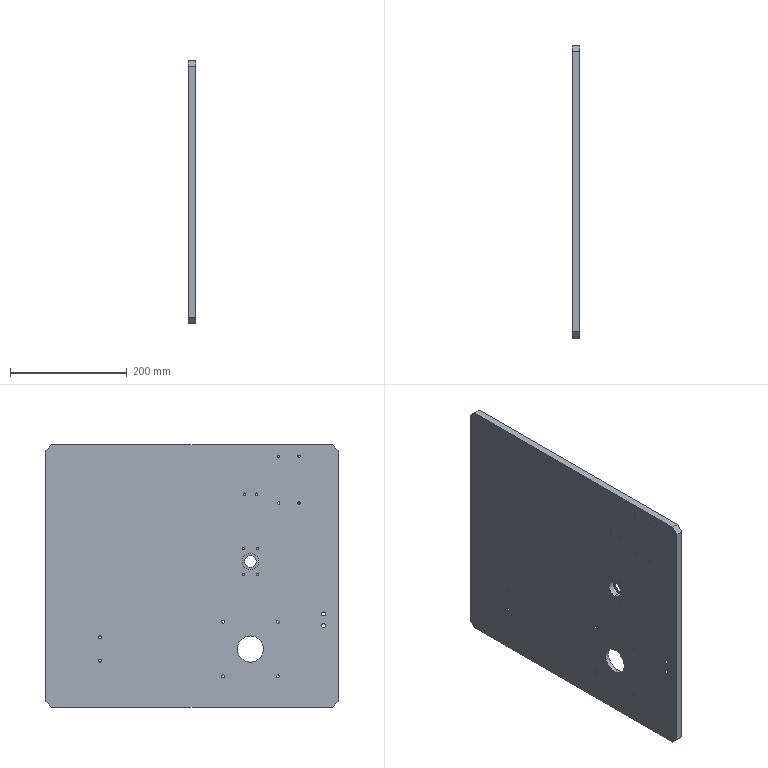Component | SolidWorks | ElectricalBoxAssembly2-1_Part6-1 | 1 solid | 56 faces | box 12 x 500 x 450 mm | volume 2647361 mm3 | cylinder 44 | plane 12 | commonest cylinder face diameters 4.2 x20 5 x12 6.8 x4 28 x2 85 x2 45 x2 20 x2
build123d program:
from build123d import *

# Parameters (mm, degrees)
SKETCH1_W            = 450
SKETCH1_H            = 500
SKETCH1_R            = 22.5
SKETCH1_R_2          = 10
BOSS_EXTRUDE1_DEPTH  = 12
M6_TAPPED_HOLE1_D    = 5
M5_TAPPED_HOLE1_D    = 4.2
M8_TAPPED_HOLE1_D    = 6.8
SKETCH9_R            = 42.5
CUT_EXTRUDE1_DEPTH   = 5
SKETCH10_R           = 14
CUT_EXTRUDE2_DEPTH   = 10
M5_TAPPED_HOLE2_D    = 4.2
M6_TAPPED_HOLE2_D    = 5
LPATTERN1_COUNT      = 2
LPATTERN1_PITCH      = 24
LPATTERN1_COUNT_DIR2 = 2
LPATTERN1_PITCH_DIR2 = 44
CHAMFER1_SIZE        = 10


with BuildPart() as part:
    # Sketch1 → Boss-Extrude1 (new body)
    with BuildSketch(Plane.XY):
        Rectangle(SKETCH1_W, SKETCH1_H)
        with Locations((125, 100)):
            Circle(SKETCH1_R, mode=Mode.SUBTRACT)
        with Locations((-25, 100)):
            Circle(SKETCH1_R_2, mode=Mode.SUBTRACT)
    extrude(amount=BOSS_EXTRUDE1_DEPTH)

    # M6 Tapped Hole1 (through all)
    with Locations(Plane.XY.offset(12)):
        with Locations((78.331, 146.669), (171.669, 146.669), (78.331, 53.331), (171.669, 53.331)):
            Hole(M6_TAPPED_HOLE1_D / 2)

    # M5 Tapped Hole1 (through all)
    with Locations(Plane.XY.offset(12)):
        with Locations((-205, 183.388), (-205, 148.388), (-125, 183.388), (-125, 148.388)):
            Hole(M5_TAPPED_HOLE1_D / 2)

    # M8 Tapped Hole1 (through all)
    with Locations(Plane.XY.offset(12)):
        with Locations((85, 225), (65, 225)):
            Hole(M8_TAPPED_HOLE1_D / 2)

    # Sketch9 → Cut-Extrude1 (cut)
    with BuildSketch(Plane(origin=(0, 0, 0), x_dir=(-1, 0, 0), z_dir=(0, 0, -1))):
        with Locations((-125, 100)):
            Circle(SKETCH9_R)
    extrude(amount=-CUT_EXTRUDE1_DEPTH, mode=Mode.SUBTRACT)

    # Sketch10 → Cut-Extrude2 (cut)
    with BuildSketch(Plane.XY.offset(12)):
        with Locations((-25, 100)):
            Circle(SKETCH10_R)
    extrude(amount=-CUT_EXTRUDE2_DEPTH, mode=Mode.SUBTRACT)

    # M5 Tapped Hole2 (through all)
    with Locations(Plane(origin=(0, 0, 0), x_dir=(-1, 0, 0), z_dir=(0, 0, -1))):
        with Locations((140, 110), (140, 90)):
            Hole(M5_TAPPED_HOLE2_D / 2)

    # M6 Tapped Hole2 (through all)
    with Locations(Plane.XY.offset(12)):
        with Locations((105, -157.5), (145, -157.5)):
            Hole(M6_TAPPED_HOLE2_D / 2)

    # Sketch16 → M5 Tapped Hole3 (revolve, cut)
    with BuildSketch(Plane(origin=(-3, 112, 0), x_dir=(0, 1, 0), z_dir=(1, 0, 0))):
        Polygon((0, 0), (0, 13.662), (2.1, 12.4), (2.1, 0), align=None)
    m5_tapped_hole3 = revolve(axis=Axis((-3, 112, -6.35), (0, 0, 1)), mode=Mode.SUBTRACT)

    # LPattern1: M5 Tapped Hole3 2 × 2
    with Locations(*[(-j * LPATTERN1_PITCH_DIR2, -i * LPATTERN1_PITCH, 0) for i in range(LPATTERN1_COUNT) for j in range(LPATTERN1_COUNT_DIR2) if (i, j) != (0, 0)]):
        add(m5_tapped_hole3, mode=Mode.SUBTRACT)

    # Chamfer1
    chamfer1_edges = [part.edges().sort_by_distance(p)[0] for p in [
        (-225, 250, 6),
        (225, 250, 6),
        (225, -250, 6),
        (-225, -250, 6),
    ]]
    chamfer(chamfer1_edges, length=CHAMFER1_SIZE)


solid = part.part

# Placed as in the assembly
solid = solid.moved(Location((767.468, 314.666, 1651.399), (180, -90, 0)))